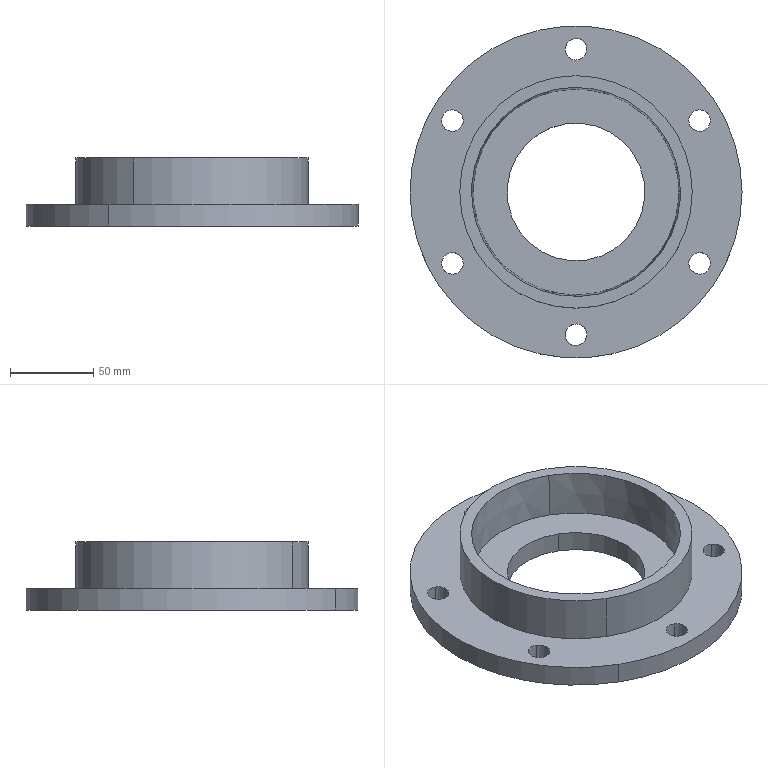Component | SolidWorks | PartAssemblyInLowerHousing-1_FlangeOnLowSpeedAxis2-1 | 1 solid | 24 faces | box 200 x 200 x 41 mm | volume 411686 mm3 | cylinder 18 | plane 4 | cone 2 | commonest cylinder face diameters 13 x12 83 x2 140 x2 200 x2
build123d program:
from build123d import *

# Parameters (mm, degrees)
SKETCH2_R          = 6.5
CUT_EXTRUDE1_DEPTH = 145.167
CIRPATTERN1_COUNT  = 6
SKETCH3_R          = 41.5
CUT_EXTRUDE2_DEPTH = 148.245
DRAFT1_ANGLE       = 2


with BuildPart() as part:
    # Sketch1 → Revolve1 (revolve)
    with BuildSketch(Plane.XY, mode=Mode.PRIVATE) as revolve1_sk:
        Polygon((0, 0), (0, 100), (13, 100), (13, 70), (41, 70), (41, 62), (12.495, 62), (12.495, 0), align=None)
    revolve(revolve1_sk.sketch.rotate(Axis((0, 0, 0), (1, 0, 0)), 90), axis=Axis((0, 0, 0), (1, 0, 0)))

    # Sketch2 → Cut-Extrude1 (cut, through all)
    with BuildSketch(Plane(origin=(13, 0, 0), x_dir=(0, 0, -1), z_dir=(1, 0, 0))):
        with Locations((0, 86)):
            Circle(SKETCH2_R)
    cut_extrude1 = extrude(amount=-CUT_EXTRUDE1_DEPTH, mode=Mode.SUBTRACT)

    # CirPattern1: Cut-Extrude1 ×6 about axis
    cirpattern1_axis = Axis((0, 0, 0), (1, 0, 0))
    for i in range(1, CIRPATTERN1_COUNT):
        add(cut_extrude1.rotate(cirpattern1_axis, i * 360 / CIRPATTERN1_COUNT), mode=Mode.SUBTRACT)

    # Sketch3 → Cut-Extrude2 (cut, through all)
    with BuildSketch(Plane.ZY):
        Circle(SKETCH3_R)
    extrude(amount=-CUT_EXTRUDE2_DEPTH, mode=Mode.SUBTRACT)

    # Draft1
    draft1_faces = [part.faces().sort_by_distance(p)[0] for p in [
        (26.748, 0, -62),
    ]]
    draft(draft1_faces, Plane(origin=(12.495, 62, 0), x_dir=(0, 0, 1), z_dir=(1, 0, 0)), DRAFT1_ANGLE)


solid = part.part

# Placed as in the assembly
solid = solid.moved(Location((1140.83, 1268.591, 1428.217), (0, -90, 0)))
STEP:
#1=COLOUR_RGB('',0.7922,0.8196,0.9333);
#2=FILL_AREA_STYLE_COLOUR('',#1);
#3=FILL_AREA_STYLE('',(#2));
#4=SURFACE_STYLE_FILL_AREA(#3);
#5=SURFACE_SIDE_STYLE('',(#4));
#6=SURFACE_STYLE_USAGE(.BOTH.,#5);
#7=PRESENTATION_STYLE_ASSIGNMENT((#6));
#8=CARTESIAN_POINT('',(45.731,51.359,56.721));
#9=VERTEX_POINT('',#8);
#10=CARTESIAN_POINT('',(44.098,48.53,56.721));
#11=VERTEX_POINT('',#10);
#12=CARTESIAN_POINT('',(44.915,49.945,56.721));
#13=DIRECTION('',(0.,0.,-1.));
#14=DIRECTION('',(-0.5,-0.866,0.));
#15=AXIS2_PLACEMENT_3D('',#12,#13,#14);
#16=CIRCLE('',#15,1.634);
#17=EDGE_CURVE('',#9,#11,#16,.T.);
#18=ORIENTED_EDGE('',*,*,#17,.F.);
#19=CARTESIAN_POINT('',(45.731,51.359,56.229));
#20=VERTEX_POINT('',#19);
#21=CARTESIAN_POINT('',(45.731,51.359,57.843));
#22=DIRECTION('',(0.,0.,-1.));
#23=VECTOR('',#22,39.37);
#24=LINE('',#21,#23);
#25=EDGE_CURVE('',#9,#20,#24,.T.);
#26=ORIENTED_EDGE('',*,*,#25,.T.);
#27=CARTESIAN_POINT('',(44.098,48.53,56.229));
#28=VERTEX_POINT('',#27);
#29=CARTESIAN_POINT('',(44.915,49.945,56.229));
#30=DIRECTION('',(0.,0.,-1.));
#31=DIRECTION('',(-0.5,-0.866,0.));
#32=AXIS2_PLACEMENT_3D('',#29,#30,#31);
#33=CIRCLE('',#32,1.634);
#34=EDGE_CURVE('',#20,#28,#33,.T.);
#35=ORIENTED_EDGE('',*,*,#34,.T.);
#36=CARTESIAN_POINT('',(44.098,48.53,57.843));
#37=DIRECTION('',(0.,0.,-1.));
#38=VECTOR('',#37,39.37);
#39=LINE('',#36,#38);
#40=EDGE_CURVE('',#11,#28,#39,.T.);
#41=ORIENTED_EDGE('',*,*,#40,.F.);
#42=EDGE_LOOP('',(#18,#26,#35,#41));
#43=FACE_OUTER_BOUND('',#42,.T.);
#44=CARTESIAN_POINT('',(44.915,49.945,57.843));
#45=DIRECTION('',(0.,0.,-1.));
#46=DIRECTION('',(-0.5,-0.866,0.));
#47=AXIS2_PLACEMENT_3D('',#44,#45,#46);
#48=CYLINDRICAL_SURFACE('',#47,1.634);
#49=ADVANCED_FACE('',(#43),#48,.F.);
#50=CARTESIAN_POINT('',(44.787,53.109,56.229));
#51=VERTEX_POINT('',#50);
#52=CARTESIAN_POINT('',(45.043,53.552,56.229));
#53=VERTEX_POINT('',#52);
#54=CARTESIAN_POINT('',(44.915,53.33,56.229));
#55=DIRECTION('',(0.,0.,1.));
#56=DIRECTION('',(1.,0.,0.));
#57=AXIS2_PLACEMENT_3D('',#54,#55,#56);
#58=CIRCLE('',#57,0.2559);
#59=EDGE_CURVE('',#51,#53,#58,.T.);
#60=ORIENTED_EDGE('',*,*,#59,.F.);
#61=CARTESIAN_POINT('',(44.787,53.109,56.741));
#62=VERTEX_POINT('',#61);
#63=CARTESIAN_POINT('',(44.787,53.109,56.229));
#64=DIRECTION('',(0.,0.,1.));
#65=VECTOR('',#64,39.37);
#66=LINE('',#63,#65);
#67=EDGE_CURVE('',#51,#62,#66,.T.);
#68=ORIENTED_EDGE('',*,*,#67,.T.);
#69=CARTESIAN_POINT('',(45.043,53.552,56.741));
#70=VERTEX_POINT('',#69);
#71=CARTESIAN_POINT('',(44.915,53.33,56.741));
#72=DIRECTION('',(0.,0.,1.));
#73=DIRECTION('',(1.,0.,0.));
#74=AXIS2_PLACEMENT_3D('',#71,#72,#73);
#75=CIRCLE('',#74,0.2559);
#76=EDGE_CURVE('',#62,#70,#75,.T.);
#77=ORIENTED_EDGE('',*,*,#76,.T.);
#78=CARTESIAN_POINT('',(45.043,53.552,56.229));
#79=DIRECTION('',(0.,0.,1.));
#80=VECTOR('',#79,39.37);
#81=LINE('',#78,#80);
#82=EDGE_CURVE('',#53,#70,#81,.T.);
#83=ORIENTED_EDGE('',*,*,#82,.F.);
#84=EDGE_LOOP('',(#60,#68,#77,#83));
#85=FACE_OUTER_BOUND('',#84,.T.);
#86=CARTESIAN_POINT('',(44.915,53.33,56.229));
#87=DIRECTION('',(0.,0.,1.));
#88=DIRECTION('',(0.5,0.866,0.));
#89=AXIS2_PLACEMENT_3D('',#86,#87,#88);
#90=CYLINDRICAL_SURFACE('',#89,0.2559);
#91=ADVANCED_FACE('',(#85),#90,.F.);
#92=CARTESIAN_POINT('',(47.719,51.416,56.229));
#93=VERTEX_POINT('',#92);
#94=CARTESIAN_POINT('',(47.975,51.859,56.229));
#95=VERTEX_POINT('',#94);
#96=CARTESIAN_POINT('',(47.847,51.637,56.229));
#97=DIRECTION('',(0.,0.,1.));
#98=DIRECTION('',(0.5,-0.866,0.));
#99=AXIS2_PLACEMENT_3D('',#96,#97,#98);
#100=CIRCLE('',#99,0.2559);
#101=EDGE_CURVE('',#93,#95,#100,.T.);
#102=ORIENTED_EDGE('',*,*,#101,.F.);
#103=CARTESIAN_POINT('',(47.719,51.416,56.741));
#104=VERTEX_POINT('',#103);
#105=CARTESIAN_POINT('',(47.719,51.416,56.229));
#106=DIRECTION('',(0.,0.,1.));
#107=VECTOR('',#106,39.37);
#108=LINE('',#105,#107);
#109=EDGE_CURVE('',#93,#104,#108,.T.);
#110=ORIENTED_EDGE('',*,*,#109,.T.);
#111=CARTESIAN_POINT('',(47.975,51.859,56.741));
#112=VERTEX_POINT('',#111);
#113=CARTESIAN_POINT('',(47.847,51.637,56.741));
#114=DIRECTION('',(0.,0.,1.));
#115=DIRECTION('',(0.5,-0.866,0.));
#116=AXIS2_PLACEMENT_3D('',#113,#114,#115);
#117=CIRCLE('',#116,0.2559);
#118=EDGE_CURVE('',#104,#112,#117,.T.);
#119=ORIENTED_EDGE('',*,*,#118,.T.);
#120=CARTESIAN_POINT('',(47.975,51.859,56.229));
#121=DIRECTION('',(0.,0.,1.));
#122=VECTOR('',#121,39.37);
#123=LINE('',#120,#122);
#124=EDGE_CURVE('',#95,#112,#123,.T.);
#125=ORIENTED_EDGE('',*,*,#124,.F.);
#126=EDGE_LOOP('',(#102,#110,#119,#125));
#127=FACE_OUTER_BOUND('',#126,.T.);
#128=CARTESIAN_POINT('',(47.847,51.637,56.229));
#129=DIRECTION('',(0.,0.,1.));
#130=DIRECTION('',(0.5,0.866,0.));
#131=AXIS2_PLACEMENT_3D('',#128,#129,#130);
#132=CYLINDRICAL_SURFACE('',#131,0.2559);
#133=ADVANCED_FACE('',(#127),#132,.F.);
#134=CARTESIAN_POINT('',(47.719,48.03,56.229));
#135=VERTEX_POINT('',#134);
#136=CARTESIAN_POINT('',(47.975,48.473,56.229));
#137=VERTEX_POINT('',#136);
#138=CARTESIAN_POINT('',(47.847,48.252,56.229));
#139=DIRECTION('',(0.,0.,1.));
#140=DIRECTION('',(-0.5,-0.866,0.));
#141=AXIS2_PLACEMENT_3D('',#138,#139,#140);
#142=CIRCLE('',#141,0.2559);
#143=EDGE_CURVE('',#135,#137,#142,.T.);
#144=ORIENTED_EDGE('',*,*,#143,.F.);
#145=CARTESIAN_POINT('',(47.719,48.03,56.741));
#146=VERTEX_POINT('',#145);
#147=CARTESIAN_POINT('',(47.719,48.03,56.229));
#148=DIRECTION('',(0.,0.,1.));
#149=VECTOR('',#148,39.37);
#150=LINE('',#147,#149);
#151=EDGE_CURVE('',#135,#146,#150,.T.);
#152=ORIENTED_EDGE('',*,*,#151,.T.);
#153=CARTESIAN_POINT('',(47.975,48.473,56.741));
#154=VERTEX_POINT('',#153);
#155=CARTESIAN_POINT('',(47.847,48.252,56.741));
#156=DIRECTION('',(0.,0.,1.));
#157=DIRECTION('',(-0.5,-0.866,0.));
#158=AXIS2_PLACEMENT_3D('',#155,#156,#157);
#159=CIRCLE('',#158,0.2559);
#160=EDGE_CURVE('',#146,#154,#159,.T.);
#161=ORIENTED_EDGE('',*,*,#160,.T.);
#162=CARTESIAN_POINT('',(47.975,48.473,56.229));
#163=DIRECTION('',(0.,0.,1.));
#164=VECTOR('',#163,39.37);
#165=LINE('',#162,#164);
#166=EDGE_CURVE('',#137,#154,#165,.T.);
#167=ORIENTED_EDGE('',*,*,#166,.F.);
#168=EDGE_LOOP('',(#144,#152,#161,#167));
#169=FACE_OUTER_BOUND('',#168,.T.);
#170=CARTESIAN_POINT('',(47.847,48.252,56.229));
#171=DIRECTION('',(0.,0.,1.));
#172=DIRECTION('',(0.5,0.866,0.));
#173=AXIS2_PLACEMENT_3D('',#170,#171,#172);
#174=CYLINDRICAL_SURFACE('',#173,0.2559);
#175=ADVANCED_FACE('',(#169),#174,.F.);
#176=CARTESIAN_POINT('',(44.787,46.337,56.229));
#177=VERTEX_POINT('',#176);
#178=CARTESIAN_POINT('',(45.043,46.78,56.229));
#179=VERTEX_POINT('',#178);
#180=CARTESIAN_POINT('',(44.915,46.559,56.229));
#181=DIRECTION('',(0.,0.,1.));
#182=DIRECTION('',(-1.,0.,0.));
#183=AXIS2_PLACEMENT_3D('',#180,#181,#182);
#184=CIRCLE('',#183,0.2559);
#185=EDGE_CURVE('',#177,#179,#184,.T.);
#186=ORIENTED_EDGE('',*,*,#185,.F.);
#187=CARTESIAN_POINT('',(44.787,46.337,56.741));
#188=VERTEX_POINT('',#187);
#189=CARTESIAN_POINT('',(44.787,46.337,56.229));
#190=DIRECTION('',(0.,0.,1.));
#191=VECTOR('',#190,39.37);
#192=LINE('',#189,#191);
#193=EDGE_CURVE('',#177,#188,#192,.T.);
#194=ORIENTED_EDGE('',*,*,#193,.T.);
#195=CARTESIAN_POINT('',(45.043,46.78,56.741));
#196=VERTEX_POINT('',#195);
#197=CARTESIAN_POINT('',(44.915,46.559,56.741));
#198=DIRECTION('',(0.,0.,1.));
#199=DIRECTION('',(-1.,0.,0.));
#200=AXIS2_PLACEMENT_3D('',#197,#198,#199);
#201=CIRCLE('',#200,0.2559);
#202=EDGE_CURVE('',#188,#196,#201,.T.);
#203=ORIENTED_EDGE('',*,*,#202,.T.);
#204=CARTESIAN_POINT('',(45.043,46.78,56.229));
#205=DIRECTION('',(0.,0.,1.));
#206=VECTOR('',#205,39.37);
#207=LINE('',#204,#206);
#208=EDGE_CURVE('',#179,#196,#207,.T.);
#209=ORIENTED_EDGE('',*,*,#208,.F.);
#210=EDGE_LOOP('',(#186,#194,#203,#209));
#211=FACE_OUTER_BOUND('',#210,.T.);
#212=CARTESIAN_POINT('',(44.915,46.559,56.229));
#213=DIRECTION('',(0.,0.,1.));
#214=DIRECTION('',(0.5,0.866,0.));
#215=AXIS2_PLACEMENT_3D('',#212,#213,#214);
#216=CYLINDRICAL_SURFACE('',#215,0.2559);
#217=ADVANCED_FACE('',(#211),#216,.F.);
#218=CARTESIAN_POINT('',(41.854,48.03,56.229));
#219=VERTEX_POINT('',#218);
#220=CARTESIAN_POINT('',(42.11,48.473,56.229));
#221=VERTEX_POINT('',#220);
#222=CARTESIAN_POINT('',(41.982,48.252,56.229));
#223=DIRECTION('',(0.,0.,1.));
#224=DIRECTION('',(-0.5,0.866,0.));
#225=AXIS2_PLACEMENT_3D('',#222,#223,#224);
#226=CIRCLE('',#225,0.2559);
#227=EDGE_CURVE('',#219,#221,#226,.T.);
#228=ORIENTED_EDGE('',*,*,#227,.F.);
#229=CARTESIAN_POINT('',(41.854,48.03,56.741));
#230=VERTEX_POINT('',#229);
#231=CARTESIAN_POINT('',(41.854,48.03,56.229));
#232=DIRECTION('',(0.,0.,1.));
#233=VECTOR('',#232,39.37);
#234=LINE('',#231,#233);
#235=EDGE_CURVE('',#219,#230,#234,.T.);
#236=ORIENTED_EDGE('',*,*,#235,.T.);
#237=CARTESIAN_POINT('',(42.11,48.473,56.741));
#238=VERTEX_POINT('',#237);
#239=CARTESIAN_POINT('',(41.982,48.252,56.741));
#240=DIRECTION('',(0.,0.,1.));
#241=DIRECTION('',(-0.5,0.866,0.));
#242=AXIS2_PLACEMENT_3D('',#239,#240,#241);
#243=CIRCLE('',#242,0.2559);
#244=EDGE_CURVE('',#230,#238,#243,.T.);
#245=ORIENTED_EDGE('',*,*,#244,.T.);
#246=CARTESIAN_POINT('',(42.11,48.473,56.229));
#247=DIRECTION('',(0.,0.,1.));
#248=VECTOR('',#247,39.37);
#249=LINE('',#246,#248);
#250=EDGE_CURVE('',#221,#238,#249,.T.);
#251=ORIENTED_EDGE('',*,*,#250,.F.);
#252=EDGE_LOOP('',(#228,#236,#245,#251));
#253=FACE_OUTER_BOUND('',#252,.T.);
#254=CARTESIAN_POINT('',(41.982,48.252,56.229));
#255=DIRECTION('',(0.,0.,1.));
#256=DIRECTION('',(0.5,0.866,0.));
#257=AXIS2_PLACEMENT_3D('',#254,#255,#256);
#258=CYLINDRICAL_SURFACE('',#257,0.2559);
#259=ADVANCED_FACE('',(#253),#258,.F.);
#260=CARTESIAN_POINT('',(41.854,51.416,56.229));
#261=VERTEX_POINT('',#260);
#262=CARTESIAN_POINT('',(42.11,51.859,56.229));
#263=VERTEX_POINT('',#262);
#264=CARTESIAN_POINT('',(41.982,51.637,56.229));
#265=DIRECTION('',(0.,0.,1.));
#266=DIRECTION('',(0.5,0.866,0.));
#267=AXIS2_PLACEMENT_3D('',#264,#265,#266);
#268=CIRCLE('',#267,0.2559);
#269=EDGE_CURVE('',#261,#263,#268,.T.);
#270=ORIENTED_EDGE('',*,*,#269,.F.);
#271=CARTESIAN_POINT('',(41.854,51.416,56.741));
#272=VERTEX_POINT('',#271);
#273=CARTESIAN_POINT('',(41.854,51.416,56.229));
#274=DIRECTION('',(0.,0.,1.));
#275=VECTOR('',#274,39.37);
#276=LINE('',#273,#275);
#277=EDGE_CURVE('',#261,#272,#276,.T.);
#278=ORIENTED_EDGE('',*,*,#277,.T.);
#279=CARTESIAN_POINT('',(42.11,51.859,56.741));
#280=VERTEX_POINT('',#279);
#281=CARTESIAN_POINT('',(41.982,51.637,56.741));
#282=DIRECTION('',(0.,0.,1.));
#283=DIRECTION('',(0.5,0.866,0.));
#284=AXIS2_PLACEMENT_3D('',#281,#282,#283);
#285=CIRCLE('',#284,0.2559);
#286=EDGE_CURVE('',#272,#280,#285,.T.);
#287=ORIENTED_EDGE('',*,*,#286,.T.);
#288=CARTESIAN_POINT('',(42.11,51.859,56.229));
#289=DIRECTION('',(0.,0.,1.));
#290=VECTOR('',#289,39.37);
#291=LINE('',#288,#290);
#292=EDGE_CURVE('',#263,#280,#291,.T.);
#293=ORIENTED_EDGE('',*,*,#292,.F.);
#294=EDGE_LOOP('',(#270,#278,#287,#293));
#295=FACE_OUTER_BOUND('',#294,.T.);
#296=CARTESIAN_POINT('',(41.982,51.637,56.229));
#297=DIRECTION('',(0.,0.,1.));
#298=DIRECTION('',(0.5,0.866,0.));
#299=AXIS2_PLACEMENT_3D('',#296,#297,#298);
#300=CYLINDRICAL_SURFACE('',#299,0.2559);
#301=ADVANCED_FACE('',(#295),#300,.F.);
#302=CARTESIAN_POINT('',(43.694,47.831,56.721));
#303=VERTEX_POINT('',#302);
#304=CARTESIAN_POINT('',(46.135,52.058,56.721));
#305=VERTEX_POINT('',#304);
#306=CARTESIAN_POINT('',(44.915,49.945,56.721));
#307=DIRECTION('',(0.,0.,-1.));
#308=DIRECTION('',(-0.5,-0.866,0.));
#309=AXIS2_PLACEMENT_3D('',#306,#307,#308);
#310=CIRCLE('',#309,2.441);
#311=EDGE_CURVE('',#303,#305,#310,.T.);
#312=ORIENTED_EDGE('',*,*,#311,.T.);
#313=CARTESIAN_POINT('',(46.155,52.092,57.843));
#314=VERTEX_POINT('',#313);
#315=CARTESIAN_POINT('',(46.135,52.058,56.721));
#316=DIRECTION('',(0.01745,0.03022,0.9994));
#317=VECTOR('',#316,39.37);
#318=LINE('',#315,#317);
#319=EDGE_CURVE('',#305,#314,#318,.T.);
#320=ORIENTED_EDGE('',*,*,#319,.T.);
#321=CARTESIAN_POINT('',(43.674,47.797,57.843));
#322=VERTEX_POINT('',#321);
#323=CARTESIAN_POINT('',(44.915,49.945,57.843));
#324=DIRECTION('',(0.,0.,-1.));
#325=DIRECTION('',(-0.5,-0.866,0.));
#326=AXIS2_PLACEMENT_3D('',#323,#324,#325);
#327=CIRCLE('',#326,2.48);
#328=EDGE_CURVE('',#322,#314,#327,.T.);
#329=ORIENTED_EDGE('',*,*,#328,.F.);
#330=CARTESIAN_POINT('',(43.694,47.831,56.721));
#331=DIRECTION('',(-0.01745,-0.03022,0.9994));
#332=VECTOR('',#331,39.37);
#333=LINE('',#330,#332);
#334=EDGE_CURVE('',#303,#322,#333,.T.);
#335=ORIENTED_EDGE('',*,*,#334,.F.);
#336=EDGE_LOOP('',(#312,#320,#329,#335));
#337=FACE_OUTER_BOUND('',#336,.T.);
#338=CARTESIAN_POINT('',(44.915,49.945,56.721));
#339=DIRECTION('',(0.,0.,1.));
#340=DIRECTION('',(-0.5,-0.866,0.));
#341=AXIS2_PLACEMENT_3D('',#338,#339,#340);
#342=CONICAL_SURFACE('',#341,2.441,0.03491);
#343=ADVANCED_FACE('',(#337),#342,.F.);
#344=CARTESIAN_POINT('',(43.537,47.558,57.843));
#345=VERTEX_POINT('',#344);
#346=CARTESIAN_POINT('',(46.293,52.331,57.843));
#347=VERTEX_POINT('',#346);
#348=CARTESIAN_POINT('',(44.915,49.945,57.843));
#349=DIRECTION('',(0.,0.,-1.));
#350=DIRECTION('',(-0.5,-0.866,0.));
#351=AXIS2_PLACEMENT_3D('',#348,#349,#350);
#352=CIRCLE('',#351,2.756);
#353=EDGE_CURVE('',#345,#347,#352,.T.);
#354=ORIENTED_EDGE('',*,*,#353,.T.);
#355=CARTESIAN_POINT('',(46.293,52.331,56.741));
#356=VERTEX_POINT('',#355);
#357=CARTESIAN_POINT('',(46.293,52.331,56.229));
#358=DIRECTION('',(0.,0.,-1.));
#359=VECTOR('',#358,39.37);
#360=LINE('',#357,#359);
#361=EDGE_CURVE('',#347,#356,#360,.T.);
#362=ORIENTED_EDGE('',*,*,#361,.T.);
#363=CARTESIAN_POINT('',(43.537,47.558,56.741));
#364=VERTEX_POINT('',#363);
#365=CARTESIAN_POINT('',(44.915,49.945,56.741));
#366=DIRECTION('',(0.,0.,-1.));
#367=DIRECTION('',(-0.5,-0.866,0.));
#368=AXIS2_PLACEMENT_3D('',#365,#366,#367);
#369=CIRCLE('',#368,2.756);
#370=EDGE_CURVE('',#364,#356,#369,.T.);
#371=ORIENTED_EDGE('',*,*,#370,.F.);
#372=CARTESIAN_POINT('',(43.537,47.558,56.229));
#373=DIRECTION('',(0.,0.,-1.));
#374=VECTOR('',#373,39.37);
#375=LINE('',#372,#374);
#376=EDGE_CURVE('',#345,#364,#375,.T.);
#377=ORIENTED_EDGE('',*,*,#376,.F.);
#378=EDGE_LOOP('',(#354,#362,#371,#377));
#379=FACE_OUTER_BOUND('',#378,.T.);
#380=CARTESIAN_POINT('',(44.915,49.945,56.229));
#381=DIRECTION('',(0.,0.,-1.));
#382=DIRECTION('',(-0.5,-0.866,0.));
#383=AXIS2_PLACEMENT_3D('',#380,#381,#382);
#384=CYLINDRICAL_SURFACE('',#383,2.756);
#385=ADVANCED_FACE('',(#379),#384,.T.);
#386=CARTESIAN_POINT('',(42.946,46.535,56.741));
#387=VERTEX_POINT('',#386);
#388=CARTESIAN_POINT('',(46.883,53.354,56.741));
#389=VERTEX_POINT('',#388);
#390=CARTESIAN_POINT('',(44.915,49.945,56.741));
#391=DIRECTION('',(0.,0.,-1.));
#392=DIRECTION('',(-0.5,-0.866,0.));
#393=AXIS2_PLACEMENT_3D('',#390,#391,#392);
#394=CIRCLE('',#393,3.937);
#395=EDGE_CURVE('',#387,#389,#394,.T.);
#396=ORIENTED_EDGE('',*,*,#395,.T.);
#397=CARTESIAN_POINT('',(46.883,53.354,56.229));
#398=VERTEX_POINT('',#397);
#399=CARTESIAN_POINT('',(46.883,53.354,56.229));
#400=DIRECTION('',(0.,0.,-1.));
#401=VECTOR('',#400,39.37);
#402=LINE('',#399,#401);
#403=EDGE_CURVE('',#389,#398,#402,.T.);
#404=ORIENTED_EDGE('',*,*,#403,.T.);
#405=CARTESIAN_POINT('',(42.946,46.535,56.229));
#406=VERTEX_POINT('',#405);
#407=CARTESIAN_POINT('',(44.915,49.945,56.229));
#408=DIRECTION('',(0.,0.,-1.));
#409=DIRECTION('',(-0.5,-0.866,0.));
#410=AXIS2_PLACEMENT_3D('',#407,#408,#409);
#411=CIRCLE('',#410,3.937);
#412=EDGE_CURVE('',#406,#398,#411,.T.);
#413=ORIENTED_EDGE('',*,*,#412,.F.);
#414=CARTESIAN_POINT('',(42.946,46.535,56.229));
#415=DIRECTION('',(0.,0.,-1.));
#416=VECTOR('',#415,39.37);
#417=LINE('',#414,#416);
#418=EDGE_CURVE('',#387,#406,#417,.T.);
#419=ORIENTED_EDGE('',*,*,#418,.F.);
#420=EDGE_LOOP('',(#396,#404,#413,#419));
#421=FACE_OUTER_BOUND('',#420,.T.);
#422=CARTESIAN_POINT('',(44.915,49.945,56.229));
#423=DIRECTION('',(0.,0.,-1.));
#424=DIRECTION('',(-0.5,-0.866,0.));
#425=AXIS2_PLACEMENT_3D('',#422,#423,#424);
#426=CYLINDRICAL_SURFACE('',#425,3.937);
#427=ADVANCED_FACE('',(#421),#426,.T.);
#428=CARTESIAN_POINT('',(44.915,49.945,56.229));
#429=DIRECTION('',(0.,0.,-1.));
#430=DIRECTION('',(-0.5,-0.866,0.));
#431=AXIS2_PLACEMENT_3D('',#428,#429,#430);
#432=CIRCLE('',#431,1.634);
#433=EDGE_CURVE('',#28,#20,#432,.T.);
#434=ORIENTED_EDGE('',*,*,#433,.F.);
#435=ORIENTED_EDGE('',*,*,#34,.F.);
#436=EDGE_LOOP('',(#434,#435));
#437=FACE_BOUND('',#436,.T.);
#438=CARTESIAN_POINT('',(44.915,53.33,56.229));
#439=DIRECTION('',(0.,0.,1.));
#440=DIRECTION('',(1.,0.,0.));
#441=AXIS2_PLACEMENT_3D('',#438,#439,#440);
#442=CIRCLE('',#441,0.2559);
#443=EDGE_CURVE('',#53,#51,#442,.T.);
#444=ORIENTED_EDGE('',*,*,#443,.T.);
#445=ORIENTED_EDGE('',*,*,#59,.T.);
#446=EDGE_LOOP('',(#444,#445));
#447=FACE_BOUND('',#446,.T.);
#448=CARTESIAN_POINT('',(47.847,51.637,56.229));
#449=DIRECTION('',(0.,0.,1.));
#450=DIRECTION('',(0.5,-0.866,0.));
#451=AXIS2_PLACEMENT_3D('',#448,#449,#450);
#452=CIRCLE('',#451,0.2559);
#453=EDGE_CURVE('',#95,#93,#452,.T.);
#454=ORIENTED_EDGE('',*,*,#453,.T.);
#455=ORIENTED_EDGE('',*,*,#101,.T.);
#456=EDGE_LOOP('',(#454,#455));
#457=FACE_BOUND('',#456,.T.);
#458=CARTESIAN_POINT('',(47.847,48.252,56.229));
#459=DIRECTION('',(0.,0.,1.));
#460=DIRECTION('',(-0.5,-0.866,0.));
#461=AXIS2_PLACEMENT_3D('',#458,#459,#460);
#462=CIRCLE('',#461,0.2559);
#463=EDGE_CURVE('',#137,#135,#462,.T.);
#464=ORIENTED_EDGE('',*,*,#463,.T.);
#465=ORIENTED_EDGE('',*,*,#143,.T.);
#466=EDGE_LOOP('',(#464,#465));
#467=FACE_BOUND('',#466,.T.);
#468=CARTESIAN_POINT('',(44.915,46.559,56.229));
#469=DIRECTION('',(0.,0.,1.));
#470=DIRECTION('',(-1.,0.,0.));
#471=AXIS2_PLACEMENT_3D('',#468,#469,#470);
#472=CIRCLE('',#471,0.2559);
#473=EDGE_CURVE('',#179,#177,#472,.T.);
#474=ORIENTED_EDGE('',*,*,#473,.T.);
#475=ORIENTED_EDGE('',*,*,#185,.T.);
#476=EDGE_LOOP('',(#474,#475));
#477=FACE_BOUND('',#476,.T.);
#478=CARTESIAN_POINT('',(41.982,48.252,56.229));
#479=DIRECTION('',(0.,0.,1.));
#480=DIRECTION('',(-0.5,0.866,0.));
#481=AXIS2_PLACEMENT_3D('',#478,#479,#480);
#482=CIRCLE('',#481,0.2559);
#483=EDGE_CURVE('',#221,#219,#482,.T.);
#484=ORIENTED_EDGE('',*,*,#483,.T.);
#485=ORIENTED_EDGE('',*,*,#227,.T.);
#486=EDGE_LOOP('',(#484,#485));
#487=FACE_BOUND('',#486,.T.);
#488=CARTESIAN_POINT('',(41.982,51.637,56.229));
#489=DIRECTION('',(0.,0.,1.));
#490=DIRECTION('',(0.5,0.866,0.));
#491=AXIS2_PLACEMENT_3D('',#488,#489,#490);
#492=CIRCLE('',#491,0.2559);
#493=EDGE_CURVE('',#263,#261,#492,.T.);
#494=ORIENTED_EDGE('',*,*,#493,.T.);
#495=ORIENTED_EDGE('',*,*,#269,.T.);
#496=EDGE_LOOP('',(#494,#495));
#497=FACE_BOUND('',#496,.T.);
#498=ORIENTED_EDGE('',*,*,#412,.T.);
#499=CARTESIAN_POINT('',(44.915,49.945,56.229));
#500=DIRECTION('',(0.,0.,-1.));
#501=DIRECTION('',(-0.5,-0.866,0.));
#502=AXIS2_PLACEMENT_3D('',#499,#500,#501);
#503=CIRCLE('',#502,3.937);
#504=EDGE_CURVE('',#398,#406,#503,.T.);
#505=ORIENTED_EDGE('',*,*,#504,.T.);
#506=EDGE_LOOP('',(#498,#505));
#507=FACE_OUTER_BOUND('',#506,.T.);
#508=CARTESIAN_POINT('',(44.915,49.945,56.229));
#509=DIRECTION('',(0.,0.,1.));
#510=DIRECTION('',(0.5,0.866,0.));
#511=AXIS2_PLACEMENT_3D('',#508,#509,#510);
#512=PLANE('',#511);
#513=ADVANCED_FACE('',(#437,#447,#457,#467,#477,#487,#497,#507),#512,.F.);
#514=ORIENTED_EDGE('',*,*,#403,.F.);
#515=CARTESIAN_POINT('',(44.915,49.945,56.741));
#516=DIRECTION('',(0.,0.,-1.));
#517=DIRECTION('',(-0.5,-0.866,0.));
#518=AXIS2_PLACEMENT_3D('',#515,#516,#517);
#519=CIRCLE('',#518,3.937);
#520=EDGE_CURVE('',#389,#387,#519,.T.);
#521=ORIENTED_EDGE('',*,*,#520,.T.);
#522=ORIENTED_EDGE('',*,*,#418,.T.);
#523=ORIENTED_EDGE('',*,*,#504,.F.);
#524=EDGE_LOOP('',(#514,#521,#522,#523));
#525=FACE_OUTER_BOUND('',#524,.T.);
#526=CARTESIAN_POINT('',(44.915,49.945,56.229));
#527=DIRECTION('',(0.,0.,-1.));
#528=DIRECTION('',(-0.5,-0.866,0.));
#529=AXIS2_PLACEMENT_3D('',#526,#527,#528);
#530=CYLINDRICAL_SURFACE('',#529,3.937);
#531=ADVANCED_FACE('',(#525),#530,.T.);
#532=CARTESIAN_POINT('',(44.915,53.33,56.741));
#533=DIRECTION('',(0.,0.,1.));
#534=DIRECTION('',(1.,0.,0.));
#535=AXIS2_PLACEMENT_3D('',#532,#533,#534);
#536=CIRCLE('',#535,0.2559);
#537=EDGE_CURVE('',#70,#62,#536,.T.);
#538=ORIENTED_EDGE('',*,*,#537,.F.);
#539=ORIENTED_EDGE('',*,*,#76,.F.);
#540=EDGE_LOOP('',(#538,#539));
#541=FACE_BOUND('',#540,.T.);
#542=CARTESIAN_POINT('',(47.847,51.637,56.741));
#543=DIRECTION('',(0.,0.,1.));
#544=DIRECTION('',(0.5,-0.866,0.));
#545=AXIS2_PLACEMENT_3D('',#542,#543,#544);
#546=CIRCLE('',#545,0.2559);
#547=EDGE_CURVE('',#112,#104,#546,.T.);
#548=ORIENTED_EDGE('',*,*,#547,.F.);
#549=ORIENTED_EDGE('',*,*,#118,.F.);
#550=EDGE_LOOP('',(#548,#549));
#551=FACE_BOUND('',#550,.T.);
#552=CARTESIAN_POINT('',(47.847,48.252,56.741));
#553=DIRECTION('',(0.,0.,1.));
#554=DIRECTION('',(-0.5,-0.866,0.));
#555=AXIS2_PLACEMENT_3D('',#552,#553,#554);
#556=CIRCLE('',#555,0.2559);
#557=EDGE_CURVE('',#154,#146,#556,.T.);
#558=ORIENTED_EDGE('',*,*,#557,.F.);
#559=ORIENTED_EDGE('',*,*,#160,.F.);
#560=EDGE_LOOP('',(#558,#559));
#561=FACE_BOUND('',#560,.T.);
#562=CARTESIAN_POINT('',(44.915,46.559,56.741));
#563=DIRECTION('',(0.,0.,1.));
#564=DIRECTION('',(-1.,0.,0.));
#565=AXIS2_PLACEMENT_3D('',#562,#563,#564);
#566=CIRCLE('',#565,0.2559);
#567=EDGE_CURVE('',#196,#188,#566,.T.);
#568=ORIENTED_EDGE('',*,*,#567,.F.);
#569=ORIENTED_EDGE('',*,*,#202,.F.);
#570=EDGE_LOOP('',(#568,#569));
#571=FACE_BOUND('',#570,.T.);
#572=CARTESIAN_POINT('',(41.982,48.252,56.741));
#573=DIRECTION('',(0.,0.,1.));
#574=DIRECTION('',(-0.5,0.866,0.));
#575=AXIS2_PLACEMENT_3D('',#572,#573,#574);
#576=CIRCLE('',#575,0.2559);
#577=EDGE_CURVE('',#238,#230,#576,.T.);
#578=ORIENTED_EDGE('',*,*,#577,.F.);
#579=ORIENTED_EDGE('',*,*,#244,.F.);
#580=EDGE_LOOP('',(#578,#579));
#581=FACE_BOUND('',#580,.T.);
#582=CARTESIAN_POINT('',(41.982,51.637,56.741));
#583=DIRECTION('',(0.,0.,1.));
#584=DIRECTION('',(0.5,0.866,0.));
#585=AXIS2_PLACEMENT_3D('',#582,#583,#584);
#586=CIRCLE('',#585,0.2559);
#587=EDGE_CURVE('',#280,#272,#586,.T.);
#588=ORIENTED_EDGE('',*,*,#587,.F.);
#589=ORIENTED_EDGE('',*,*,#286,.F.);
#590=EDGE_LOOP('',(#588,#589));
#591=FACE_BOUND('',#590,.T.);
#592=ORIENTED_EDGE('',*,*,#395,.F.);
#593=ORIENTED_EDGE('',*,*,#520,.F.);
#594=EDGE_LOOP('',(#592,#593));
#595=FACE_OUTER_BOUND('',#594,.T.);
#596=ORIENTED_EDGE('',*,*,#370,.T.);
#597=CARTESIAN_POINT('',(44.915,49.945,56.741));
#598=DIRECTION('',(0.,0.,-1.));
#599=DIRECTION('',(-0.5,-0.866,0.));
#600=AXIS2_PLACEMENT_3D('',#597,#598,#599);
#601=CIRCLE('',#600,2.756);
#602=EDGE_CURVE('',#356,#364,#601,.T.);
#603=ORIENTED_EDGE('',*,*,#602,.T.);
#604=EDGE_LOOP('',(#596,#603));
#605=FACE_BOUND('',#604,.T.);
#606=CARTESIAN_POINT('',(41.505,51.913,56.741));
#607=DIRECTION('',(0.,0.,-1.));
#608=DIRECTION('',(-0.5,-0.866,0.));
#609=AXIS2_PLACEMENT_3D('',#606,#607,#608);
#610=PLANE('',#609);
#611=ADVANCED_FACE('',(#541,#551,#561,#571,#581,#591,#595,#605),#610,.F.);
#612=ORIENTED_EDGE('',*,*,#361,.F.);
#613=CARTESIAN_POINT('',(44.915,49.945,57.843));
#614=DIRECTION('',(0.,0.,-1.));
#615=DIRECTION('',(-0.5,-0.866,0.));
#616=AXIS2_PLACEMENT_3D('',#613,#614,#615);
#617=CIRCLE('',#616,2.756);
#618=EDGE_CURVE('',#347,#345,#617,.T.);
#619=ORIENTED_EDGE('',*,*,#618,.T.);
#620=ORIENTED_EDGE('',*,*,#376,.T.);
#621=ORIENTED_EDGE('',*,*,#602,.F.);
#622=EDGE_LOOP('',(#612,#619,#620,#621));
#623=FACE_OUTER_BOUND('',#622,.T.);
#624=CARTESIAN_POINT('',(44.915,49.945,56.229));
#625=DIRECTION('',(0.,0.,-1.));
#626=DIRECTION('',(-0.5,-0.866,0.));
#627=AXIS2_PLACEMENT_3D('',#624,#625,#626);
#628=CYLINDRICAL_SURFACE('',#627,2.756);
#629=ADVANCED_FACE('',(#623),#628,.T.);
#630=ORIENTED_EDGE('',*,*,#353,.F.);
#631=ORIENTED_EDGE('',*,*,#618,.F.);
#632=EDGE_LOOP('',(#630,#631));
#633=FACE_OUTER_BOUND('',#632,.T.);
#634=ORIENTED_EDGE('',*,*,#328,.T.);
#635=CARTESIAN_POINT('',(44.915,49.945,57.843));
#636=DIRECTION('',(0.,0.,-1.));
#637=DIRECTION('',(-0.5,-0.866,0.));
#638=AXIS2_PLACEMENT_3D('',#635,#636,#637);
#639=CIRCLE('',#638,2.48);
#640=EDGE_CURVE('',#314,#322,#639,.T.);
#641=ORIENTED_EDGE('',*,*,#640,.T.);
#642=EDGE_LOOP('',(#634,#641));
#643=FACE_BOUND('',#642,.T.);
#644=CARTESIAN_POINT('',(42.528,51.322,57.843));
#645=DIRECTION('',(0.,0.,-1.));
#646=DIRECTION('',(-0.5,-0.866,0.));
#647=AXIS2_PLACEMENT_3D('',#644,#645,#646);
#648=PLANE('',#647);
#649=ADVANCED_FACE('',(#633,#643),#648,.F.);
#650=ORIENTED_EDGE('',*,*,#319,.F.);
#651=CARTESIAN_POINT('',(44.915,49.945,56.721));
#652=DIRECTION('',(0.,0.,-1.));
#653=DIRECTION('',(-0.5,-0.866,0.));
#654=AXIS2_PLACEMENT_3D('',#651,#652,#653);
#655=CIRCLE('',#654,2.441);
#656=EDGE_CURVE('',#305,#303,#655,.T.);
#657=ORIENTED_EDGE('',*,*,#656,.T.);
#658=ORIENTED_EDGE('',*,*,#334,.T.);
#659=ORIENTED_EDGE('',*,*,#640,.F.);
#660=EDGE_LOOP('',(#650,#657,#658,#659));
#661=FACE_OUTER_BOUND('',#660,.T.);
#662=CARTESIAN_POINT('',(44.915,49.945,56.721));
#663=DIRECTION('',(0.,0.,1.));
#664=DIRECTION('',(-0.5,-0.866,0.));
#665=AXIS2_PLACEMENT_3D('',#662,#663,#664);
#666=CONICAL_SURFACE('',#665,2.441,0.03491);
#667=ADVANCED_FACE('',(#661),#666,.F.);
#668=CARTESIAN_POINT('',(44.915,49.945,56.721));
#669=DIRECTION('',(0.,0.,-1.));
#670=DIRECTION('',(-0.5,-0.866,0.));
#671=AXIS2_PLACEMENT_3D('',#668,#669,#670);
#672=CIRCLE('',#671,1.634);
#673=EDGE_CURVE('',#11,#9,#672,.T.);
#674=ORIENTED_EDGE('',*,*,#673,.T.);
#675=ORIENTED_EDGE('',*,*,#17,.T.);
#676=EDGE_LOOP('',(#674,#675));
#677=FACE_BOUND('',#676,.T.);
#678=ORIENTED_EDGE('',*,*,#311,.F.);
#679=ORIENTED_EDGE('',*,*,#656,.F.);
#680=EDGE_LOOP('',(#678,#679));
#681=FACE_OUTER_BOUND('',#680,.T.);
#682=CARTESIAN_POINT('',(42.801,51.165,56.721));
#683=DIRECTION('',(0.,0.,-1.));
#684=DIRECTION('',(-0.5,-0.866,0.));
#685=AXIS2_PLACEMENT_3D('',#682,#683,#684);
#686=PLANE('',#685);
#687=ADVANCED_FACE('',(#677,#681),#686,.F.);
#688=ORIENTED_EDGE('',*,*,#277,.F.);
#689=ORIENTED_EDGE('',*,*,#493,.F.);
#690=ORIENTED_EDGE('',*,*,#292,.T.);
#691=ORIENTED_EDGE('',*,*,#587,.T.);
#692=EDGE_LOOP('',(#688,#689,#690,#691));
#693=FACE_OUTER_BOUND('',#692,.T.);
#694=CARTESIAN_POINT('',(41.982,51.637,56.229));
#695=DIRECTION('',(0.,0.,1.));
#696=DIRECTION('',(0.5,0.866,0.));
#697=AXIS2_PLACEMENT_3D('',#694,#695,#696);
#698=CYLINDRICAL_SURFACE('',#697,0.2559);
#699=ADVANCED_FACE('',(#693),#698,.F.);
#700=ORIENTED_EDGE('',*,*,#235,.F.);
#701=ORIENTED_EDGE('',*,*,#483,.F.);
#702=ORIENTED_EDGE('',*,*,#250,.T.);
#703=ORIENTED_EDGE('',*,*,#577,.T.);
#704=EDGE_LOOP('',(#700,#701,#702,#703));
#705=FACE_OUTER_BOUND('',#704,.T.);
#706=CARTESIAN_POINT('',(41.982,48.252,56.229));
#707=DIRECTION('',(0.,0.,1.));
#708=DIRECTION('',(0.5,0.866,0.));
#709=AXIS2_PLACEMENT_3D('',#706,#707,#708);
#710=CYLINDRICAL_SURFACE('',#709,0.2559);
#711=ADVANCED_FACE('',(#705),#710,.F.);
#712=ORIENTED_EDGE('',*,*,#193,.F.);
#713=ORIENTED_EDGE('',*,*,#473,.F.);
#714=ORIENTED_EDGE('',*,*,#208,.T.);
#715=ORIENTED_EDGE('',*,*,#567,.T.);
#716=EDGE_LOOP('',(#712,#713,#714,#715));
#717=FACE_OUTER_BOUND('',#716,.T.);
#718=CARTESIAN_POINT('',(44.915,46.559,56.229));
#719=DIRECTION('',(0.,0.,1.));
#720=DIRECTION('',(0.5,0.866,0.));
#721=AXIS2_PLACEMENT_3D('',#718,#719,#720);
#722=CYLINDRICAL_SURFACE('',#721,0.2559);
#723=ADVANCED_FACE('',(#717),#722,.F.);
#724=ORIENTED_EDGE('',*,*,#151,.F.);
#725=ORIENTED_EDGE('',*,*,#463,.F.);
#726=ORIENTED_EDGE('',*,*,#166,.T.);
#727=ORIENTED_EDGE('',*,*,#557,.T.);
#728=EDGE_LOOP('',(#724,#725,#726,#727));
#729=FACE_OUTER_BOUND('',#728,.T.);
#730=CARTESIAN_POINT('',(47.847,48.252,56.229));
#731=DIRECTION('',(0.,0.,1.));
#732=DIRECTION('',(0.5,0.866,0.));
#733=AXIS2_PLACEMENT_3D('',#730,#731,#732);
#734=CYLINDRICAL_SURFACE('',#733,0.2559);
#735=ADVANCED_FACE('',(#729),#734,.F.);
#736=ORIENTED_EDGE('',*,*,#109,.F.);
#737=ORIENTED_EDGE('',*,*,#453,.F.);
#738=ORIENTED_EDGE('',*,*,#124,.T.);
#739=ORIENTED_EDGE('',*,*,#547,.T.);
#740=EDGE_LOOP('',(#736,#737,#738,#739));
#741=FACE_OUTER_BOUND('',#740,.T.);
#742=CARTESIAN_POINT('',(47.847,51.637,56.229));
#743=DIRECTION('',(0.,0.,1.));
#744=DIRECTION('',(0.5,0.866,0.));
#745=AXIS2_PLACEMENT_3D('',#742,#743,#744);
#746=CYLINDRICAL_SURFACE('',#745,0.2559);
#747=ADVANCED_FACE('',(#741),#746,.F.);
#748=ORIENTED_EDGE('',*,*,#67,.F.);
#749=ORIENTED_EDGE('',*,*,#443,.F.);
#750=ORIENTED_EDGE('',*,*,#82,.T.);
#751=ORIENTED_EDGE('',*,*,#537,.T.);
#752=EDGE_LOOP('',(#748,#749,#750,#751));
#753=FACE_OUTER_BOUND('',#752,.T.);
#754=CARTESIAN_POINT('',(44.915,53.33,56.229));
#755=DIRECTION('',(0.,0.,1.));
#756=DIRECTION('',(0.5,0.866,0.));
#757=AXIS2_PLACEMENT_3D('',#754,#755,#756);
#758=CYLINDRICAL_SURFACE('',#757,0.2559);
#759=ADVANCED_FACE('',(#753),#758,.F.);
#760=ORIENTED_EDGE('',*,*,#25,.F.);
#761=ORIENTED_EDGE('',*,*,#673,.F.);
#762=ORIENTED_EDGE('',*,*,#40,.T.);
#763=ORIENTED_EDGE('',*,*,#433,.T.);
#764=EDGE_LOOP('',(#760,#761,#762,#763));
#765=FACE_OUTER_BOUND('',#764,.T.);
#766=CARTESIAN_POINT('',(44.915,49.945,57.843));
#767=DIRECTION('',(0.,0.,-1.));
#768=DIRECTION('',(-0.5,-0.866,0.));
#769=AXIS2_PLACEMENT_3D('',#766,#767,#768);
#770=CYLINDRICAL_SURFACE('',#769,1.634);
#771=ADVANCED_FACE('',(#765),#770,.F.);
#772=CLOSED_SHELL('',(#49,#91,#133,#175,#217,#259,#301,#343,#385,#427,#513,#531,#611,#629,#649,#667,#687,#699,#711,#723,#735,#747,#759,#771));
#773=MANIFOLD_SOLID_BREP('',#772);
#774=STYLED_ITEM('',(#7),#773);
#775=(LENGTH_UNIT()NAMED_UNIT(*)SI_UNIT($,.METRE.));
#776=LENGTH_MEASURE_WITH_UNIT(LENGTH_MEASURE(0.0254),#775);
#777=DIMENSIONAL_EXPONENTS(1.,0.,0.,0.,0.,0.,0.);
#778=(CONVERSION_BASED_UNIT('',#776)LENGTH_UNIT()NAMED_UNIT(#777));
#779=UNCERTAINTY_MEASURE_WITH_UNIT(LENGTH_MEASURE(0.00001),#778,'','');
#780=(NAMED_UNIT(*)PLANE_ANGLE_UNIT()SI_UNIT($,.RADIAN.));
#781=(NAMED_UNIT(*)SI_UNIT($,.STERADIAN.)SOLID_ANGLE_UNIT());
#782=(GEOMETRIC_REPRESENTATION_CONTEXT(3)GLOBAL_UNCERTAINTY_ASSIGNED_CONTEXT((#779))GLOBAL_UNIT_ASSIGNED_CONTEXT((#778,#780,#781))REPRESENTATION_CONTEXT('',''));
#783=MECHANICAL_DESIGN_GEOMETRIC_PRESENTATION_REPRESENTATION('',(#774),#782);
#784=CARTESIAN_POINT('',(0.,0.,0.));
#785=DIRECTION('',(0.,0.,1.));
#786=DIRECTION('',(1.,0.,0.));
#787=AXIS2_PLACEMENT_3D('',#784,#785,#786);
#788=(LENGTH_UNIT()NAMED_UNIT(*)SI_UNIT($,.METRE.));
#789=LENGTH_MEASURE_WITH_UNIT(LENGTH_MEASURE(0.0254),#788);
#790=DIMENSIONAL_EXPONENTS(1.,0.,0.,0.,0.,0.,0.);
#791=(CONVERSION_BASED_UNIT('',#789)LENGTH_UNIT()NAMED_UNIT(#790));
#792=UNCERTAINTY_MEASURE_WITH_UNIT(LENGTH_MEASURE(0.00001),#791,'','');
#793=(NAMED_UNIT(*)PLANE_ANGLE_UNIT()SI_UNIT($,.RADIAN.));
#794=(NAMED_UNIT(*)SI_UNIT($,.STERADIAN.)SOLID_ANGLE_UNIT());
#795=(GEOMETRIC_REPRESENTATION_CONTEXT(3)GLOBAL_UNCERTAINTY_ASSIGNED_CONTEXT((#792))GLOBAL_UNIT_ASSIGNED_CONTEXT((#791,#793,#794))REPRESENTATION_CONTEXT('',''));
#796=ADVANCED_BREP_SHAPE_REPRESENTATION('',(#773,#787),#795);
#797=PRESENTATION_LAYER_ASSIGNMENT('','',(#774));